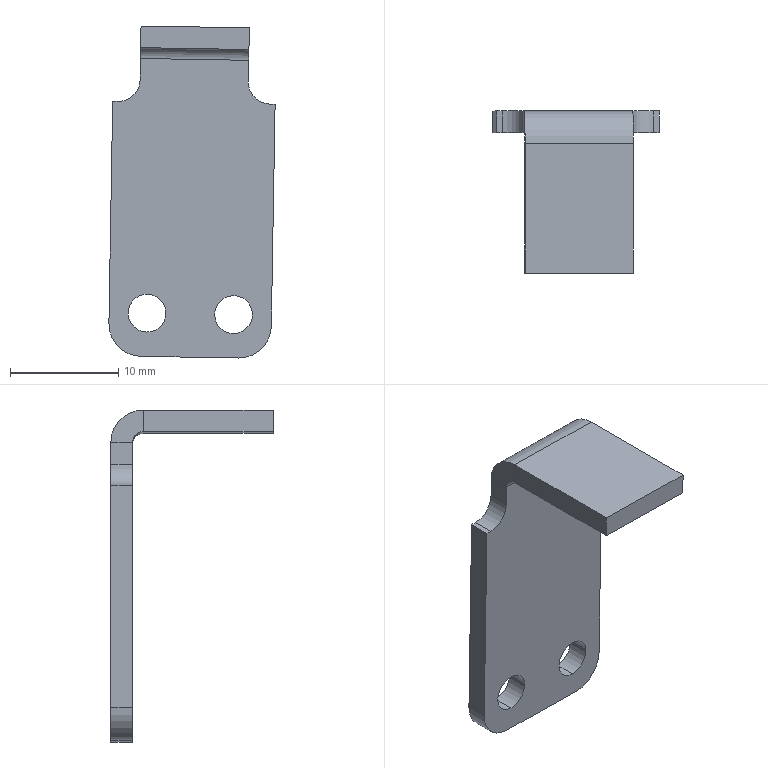Component | SolidWorks | RR40-1_InductionPlate-1 | 1 solid | 26 faces | box 15.35 x 15 x 30.66 mm | volume 1045 mm3 | plane 16 | cylinder 10 | commonest cylinder face diameters 3.5 x4 6 x3 4 x2 2 x1
STEP:
#1=COLOUR_RGB('',0.7922,0.8196,0.9333);
#2=FILL_AREA_STYLE_COLOUR('',#1);
#3=FILL_AREA_STYLE('',(#2));
#4=SURFACE_STYLE_FILL_AREA(#3);
#5=SURFACE_SIDE_STYLE('',(#4));
#6=SURFACE_STYLE_USAGE(.BOTH.,#5);
#7=PRESENTATION_STYLE_ASSIGNMENT((#6));
#8=CARTESIAN_POINT('',(22.955,37.638,-80.989));
#9=VERTEX_POINT('',#8);
#10=CARTESIAN_POINT('',(22.952,37.638,-81.127));
#11=VERTEX_POINT('',#10);
#12=CARTESIAN_POINT('',(22.953,37.638,-81.058));
#13=DIRECTION('',(-0.,-1.,-0.));
#14=DIRECTION('',(-0.01698,0.,-0.9999));
#15=AXIS2_PLACEMENT_3D('',#12,#13,#14);
#16=CIRCLE('',#15,0.0689);
#17=EDGE_CURVE('',#9,#11,#16,.T.);
#18=ORIENTED_EDGE('',*,*,#17,.T.);
#19=CARTESIAN_POINT('',(22.952,37.717,-81.127));
#20=VERTEX_POINT('',#19);
#21=CARTESIAN_POINT('',(22.952,37.717,-81.127));
#22=DIRECTION('',(0.,1.,0.));
#23=VECTOR('',#22,39.37);
#24=LINE('',#21,#23);
#25=EDGE_CURVE('',#11,#20,#24,.T.);
#26=ORIENTED_EDGE('',*,*,#25,.T.);
#27=CARTESIAN_POINT('',(22.955,37.717,-80.989));
#28=VERTEX_POINT('',#27);
#29=CARTESIAN_POINT('',(22.953,37.717,-81.058));
#30=DIRECTION('',(0.,1.,0.));
#31=DIRECTION('',(0.01698,0.,0.9999));
#32=AXIS2_PLACEMENT_3D('',#29,#30,#31);
#33=CIRCLE('',#32,0.0689);
#34=EDGE_CURVE('',#20,#28,#33,.T.);
#35=ORIENTED_EDGE('',*,*,#34,.T.);
#36=CARTESIAN_POINT('',(22.955,37.717,-80.989));
#37=DIRECTION('',(0.,1.,0.));
#38=VECTOR('',#37,39.37);
#39=LINE('',#36,#38);
#40=EDGE_CURVE('',#9,#28,#39,.T.);
#41=ORIENTED_EDGE('',*,*,#40,.F.);
#42=EDGE_LOOP('',(#18,#26,#35,#41));
#43=FACE_OUTER_BOUND('',#42,.T.);
#44=CARTESIAN_POINT('',(22.953,37.717,-81.058));
#45=DIRECTION('',(0.,1.,0.));
#46=DIRECTION('',(0.01698,0.,0.9999));
#47=AXIS2_PLACEMENT_3D('',#44,#45,#46);
#48=CYLINDRICAL_SURFACE('',#47,0.0689);
#49=ADVANCED_FACE('',(#43),#48,.F.);
#50=CARTESIAN_POINT('',(23.269,37.638,-80.994));
#51=VERTEX_POINT('',#50);
#52=CARTESIAN_POINT('',(23.267,37.638,-81.132));
#53=VERTEX_POINT('',#52);
#54=CARTESIAN_POINT('',(23.268,37.638,-81.063));
#55=DIRECTION('',(-0.,-1.,-0.));
#56=DIRECTION('',(-0.01698,0.,-0.9999));
#57=AXIS2_PLACEMENT_3D('',#54,#55,#56);
#58=CIRCLE('',#57,0.0689);
#59=EDGE_CURVE('',#51,#53,#58,.T.);
#60=ORIENTED_EDGE('',*,*,#59,.T.);
#61=CARTESIAN_POINT('',(23.267,37.717,-81.132));
#62=VERTEX_POINT('',#61);
#63=CARTESIAN_POINT('',(23.267,37.717,-81.132));
#64=DIRECTION('',(0.,1.,0.));
#65=VECTOR('',#64,39.37);
#66=LINE('',#63,#65);
#67=EDGE_CURVE('',#53,#62,#66,.T.);
#68=ORIENTED_EDGE('',*,*,#67,.T.);
#69=CARTESIAN_POINT('',(23.269,37.717,-80.994));
#70=VERTEX_POINT('',#69);
#71=CARTESIAN_POINT('',(23.268,37.717,-81.063));
#72=DIRECTION('',(0.,1.,0.));
#73=DIRECTION('',(0.01698,0.,0.9999));
#74=AXIS2_PLACEMENT_3D('',#71,#72,#73);
#75=CIRCLE('',#74,0.0689);
#76=EDGE_CURVE('',#62,#70,#75,.T.);
#77=ORIENTED_EDGE('',*,*,#76,.T.);
#78=CARTESIAN_POINT('',(23.269,37.717,-80.994));
#79=DIRECTION('',(0.,1.,0.));
#80=VECTOR('',#79,39.37);
#81=LINE('',#78,#80);
#82=EDGE_CURVE('',#51,#70,#81,.T.);
#83=ORIENTED_EDGE('',*,*,#82,.F.);
#84=EDGE_LOOP('',(#60,#68,#77,#83));
#85=FACE_OUTER_BOUND('',#84,.T.);
#86=CARTESIAN_POINT('',(23.268,37.717,-81.063));
#87=DIRECTION('',(0.,1.,0.));
#88=DIRECTION('',(0.01698,0.,0.9999));
#89=AXIS2_PLACEMENT_3D('',#86,#87,#88);
#90=CYLINDRICAL_SURFACE('',#89,0.0689);
#91=ADVANCED_FACE('',(#85),#90,.F.);
#92=CARTESIAN_POINT('',(23.323,37.638,-80.139));
#93=VERTEX_POINT('',#92);
#94=CARTESIAN_POINT('',(23.322,37.638,-80.218));
#95=VERTEX_POINT('',#94);
#96=CARTESIAN_POINT('',(23.305,37.638,-81.221));
#97=DIRECTION('',(-0.01698,0.,-0.9999));
#98=VECTOR('',#97,39.37);
#99=LINE('',#96,#98);
#100=EDGE_CURVE('',#93,#95,#99,.T.);
#101=ORIENTED_EDGE('',*,*,#100,.T.);
#102=CARTESIAN_POINT('',(23.322,37.717,-80.218));
#103=VERTEX_POINT('',#102);
#104=CARTESIAN_POINT('',(23.322,37.126,-80.218));
#105=DIRECTION('',(0.,1.,0.));
#106=VECTOR('',#105,39.37);
#107=LINE('',#104,#106);
#108=EDGE_CURVE('',#95,#103,#107,.T.);
#109=ORIENTED_EDGE('',*,*,#108,.T.);
#110=CARTESIAN_POINT('',(23.323,37.717,-80.139));
#111=VERTEX_POINT('',#110);
#112=CARTESIAN_POINT('',(23.321,37.717,-80.296));
#113=DIRECTION('',(0.01698,-0.,0.9999));
#114=VECTOR('',#113,39.37);
#115=LINE('',#112,#114);
#116=EDGE_CURVE('',#103,#111,#115,.T.);
#117=ORIENTED_EDGE('',*,*,#116,.T.);
#118=CARTESIAN_POINT('',(23.323,37.717,-80.139));
#119=DIRECTION('',(0.,-1.,0.));
#120=VECTOR('',#119,39.37);
#121=LINE('',#118,#120);
#122=EDGE_CURVE('',#111,#93,#121,.T.);
#123=ORIENTED_EDGE('',*,*,#122,.T.);
#124=EDGE_LOOP('',(#101,#109,#117,#123));
#125=FACE_OUTER_BOUND('',#124,.T.);
#126=CARTESIAN_POINT('',(23.321,37.126,-80.296));
#127=DIRECTION('',(-0.9999,0.,0.01698));
#128=DIRECTION('',(0.01698,0.,0.9999));
#129=AXIS2_PLACEMENT_3D('',#126,#127,#128);
#130=PLANE('',#129);
#131=ADVANCED_FACE('',(#125),#130,.F.);
#132=CARTESIAN_POINT('',(23.324,37.126,-80.099));
#133=VERTEX_POINT('',#132);
#134=CARTESIAN_POINT('',(23.324,37.598,-80.099));
#135=VERTEX_POINT('',#134);
#136=CARTESIAN_POINT('',(23.324,37.598,-80.099));
#137=DIRECTION('',(0.,1.,-0.));
#138=VECTOR('',#137,39.37);
#139=LINE('',#136,#138);
#140=EDGE_CURVE('',#133,#135,#139,.T.);
#141=ORIENTED_EDGE('',*,*,#140,.T.);
#142=CARTESIAN_POINT('',(23.325,37.598,-80.021));
#143=VERTEX_POINT('',#142);
#144=CARTESIAN_POINT('',(23.324,37.598,-80.099));
#145=DIRECTION('',(0.01698,0.,0.9999));
#146=VECTOR('',#145,39.37);
#147=LINE('',#144,#146);
#148=EDGE_CURVE('',#135,#143,#147,.T.);
#149=ORIENTED_EDGE('',*,*,#148,.T.);
#150=CARTESIAN_POINT('',(23.325,37.126,-80.021));
#151=VERTEX_POINT('',#150);
#152=CARTESIAN_POINT('',(23.325,37.598,-80.021));
#153=DIRECTION('',(0.,1.,-0.));
#154=VECTOR('',#153,39.37);
#155=LINE('',#152,#154);
#156=EDGE_CURVE('',#151,#143,#155,.T.);
#157=ORIENTED_EDGE('',*,*,#156,.F.);
#158=CARTESIAN_POINT('',(23.321,37.126,-80.296));
#159=DIRECTION('',(0.01698,-0.,0.9999));
#160=VECTOR('',#159,39.37);
#161=LINE('',#158,#160);
#162=EDGE_CURVE('',#133,#151,#161,.T.);
#163=ORIENTED_EDGE('',*,*,#162,.F.);
#164=EDGE_LOOP('',(#141,#149,#157,#163));
#165=FACE_OUTER_BOUND('',#164,.T.);
#166=CARTESIAN_POINT('',(23.321,37.126,-80.296));
#167=DIRECTION('',(-0.9999,0.,0.01698));
#168=DIRECTION('',(0.01698,0.,0.9999));
#169=AXIS2_PLACEMENT_3D('',#166,#167,#168);
#170=PLANE('',#169);
#171=ADVANCED_FACE('',(#165),#170,.F.);
#172=CARTESIAN_POINT('',(22.928,37.717,-80.211));
#173=VERTEX_POINT('',#172);
#174=CARTESIAN_POINT('',(22.93,37.717,-80.132));
#175=VERTEX_POINT('',#174);
#176=CARTESIAN_POINT('',(22.911,37.717,-81.215));
#177=DIRECTION('',(0.01698,-0.,0.9999));
#178=VECTOR('',#177,39.37);
#179=LINE('',#176,#178);
#180=EDGE_CURVE('',#173,#175,#179,.T.);
#181=ORIENTED_EDGE('',*,*,#180,.F.);
#182=CARTESIAN_POINT('',(22.928,37.638,-80.211));
#183=VERTEX_POINT('',#182);
#184=CARTESIAN_POINT('',(22.928,37.126,-80.211));
#185=DIRECTION('',(-0.,-1.,-0.));
#186=VECTOR('',#185,39.37);
#187=LINE('',#184,#186);
#188=EDGE_CURVE('',#173,#183,#187,.T.);
#189=ORIENTED_EDGE('',*,*,#188,.T.);
#190=CARTESIAN_POINT('',(22.93,37.638,-80.132));
#191=VERTEX_POINT('',#190);
#192=CARTESIAN_POINT('',(22.911,37.638,-81.215));
#193=DIRECTION('',(-0.01698,0.,-0.9999));
#194=VECTOR('',#193,39.37);
#195=LINE('',#192,#194);
#196=EDGE_CURVE('',#191,#183,#195,.T.);
#197=ORIENTED_EDGE('',*,*,#196,.F.);
#198=CARTESIAN_POINT('',(22.93,37.638,-80.132));
#199=DIRECTION('',(0.,1.,-0.));
#200=VECTOR('',#199,39.37);
#201=LINE('',#198,#200);
#202=EDGE_CURVE('',#191,#175,#201,.T.);
#203=ORIENTED_EDGE('',*,*,#202,.T.);
#204=EDGE_LOOP('',(#181,#189,#197,#203));
#205=FACE_OUTER_BOUND('',#204,.T.);
#206=CARTESIAN_POINT('',(22.911,37.126,-81.215));
#207=DIRECTION('',(-0.9999,0.,0.01698));
#208=DIRECTION('',(0.01698,0.,0.9999));
#209=AXIS2_PLACEMENT_3D('',#206,#207,#208);
#210=PLANE('',#209);
#211=ADVANCED_FACE('',(#205),#210,.T.);
#212=CARTESIAN_POINT('',(22.932,37.126,-80.014));
#213=VERTEX_POINT('',#212);
#214=CARTESIAN_POINT('',(22.932,37.598,-80.014));
#215=VERTEX_POINT('',#214);
#216=CARTESIAN_POINT('',(22.932,37.598,-80.014));
#217=DIRECTION('',(0.,1.,-0.));
#218=VECTOR('',#217,39.37);
#219=LINE('',#216,#218);
#220=EDGE_CURVE('',#213,#215,#219,.T.);
#221=ORIENTED_EDGE('',*,*,#220,.T.);
#222=CARTESIAN_POINT('',(22.93,37.598,-80.093));
#223=VERTEX_POINT('',#222);
#224=CARTESIAN_POINT('',(22.932,37.598,-80.014));
#225=DIRECTION('',(-0.01698,-0.,-0.9999));
#226=VECTOR('',#225,39.37);
#227=LINE('',#224,#226);
#228=EDGE_CURVE('',#215,#223,#227,.T.);
#229=ORIENTED_EDGE('',*,*,#228,.T.);
#230=CARTESIAN_POINT('',(22.93,37.126,-80.093));
#231=VERTEX_POINT('',#230);
#232=CARTESIAN_POINT('',(22.93,37.598,-80.093));
#233=DIRECTION('',(0.,1.,-0.));
#234=VECTOR('',#233,39.37);
#235=LINE('',#232,#234);
#236=EDGE_CURVE('',#231,#223,#235,.T.);
#237=ORIENTED_EDGE('',*,*,#236,.F.);
#238=CARTESIAN_POINT('',(22.911,37.126,-81.215));
#239=DIRECTION('',(0.01698,-0.,0.9999));
#240=VECTOR('',#239,39.37);
#241=LINE('',#238,#240);
#242=EDGE_CURVE('',#231,#213,#241,.T.);
#243=ORIENTED_EDGE('',*,*,#242,.T.);
#244=EDGE_LOOP('',(#221,#229,#237,#243));
#245=FACE_OUTER_BOUND('',#244,.T.);
#246=CARTESIAN_POINT('',(22.911,37.126,-81.215));
#247=DIRECTION('',(-0.9999,0.,0.01698));
#248=DIRECTION('',(0.01698,0.,0.9999));
#249=AXIS2_PLACEMENT_3D('',#246,#247,#248);
#250=PLANE('',#249);
#251=ADVANCED_FACE('',(#245),#250,.T.);
#252=ORIENTED_EDGE('',*,*,#17,.F.);
#253=CARTESIAN_POINT('',(22.953,37.638,-81.058));
#254=DIRECTION('',(-0.,-1.,-0.));
#255=DIRECTION('',(-0.01698,0.,-0.9999));
#256=AXIS2_PLACEMENT_3D('',#253,#254,#255);
#257=CIRCLE('',#256,0.0689);
#258=EDGE_CURVE('',#11,#9,#257,.T.);
#259=ORIENTED_EDGE('',*,*,#258,.F.);
#260=EDGE_LOOP('',(#252,#259));
#261=FACE_BOUND('',#260,.T.);
#262=ORIENTED_EDGE('',*,*,#59,.F.);
#263=CARTESIAN_POINT('',(23.268,37.638,-81.063));
#264=DIRECTION('',(-0.,-1.,-0.));
#265=DIRECTION('',(-0.01698,0.,-0.9999));
#266=AXIS2_PLACEMENT_3D('',#263,#264,#265);
#267=CIRCLE('',#266,0.0689);
#268=EDGE_CURVE('',#53,#51,#267,.T.);
#269=ORIENTED_EDGE('',*,*,#268,.F.);
#270=EDGE_LOOP('',(#262,#269));
#271=FACE_BOUND('',#270,.T.);
#272=CARTESIAN_POINT('',(23.405,37.638,-81.105));
#273=VERTEX_POINT('',#272);
#274=CARTESIAN_POINT('',(23.419,37.638,-80.298));
#275=VERTEX_POINT('',#274);
#276=CARTESIAN_POINT('',(23.403,37.638,-81.223));
#277=DIRECTION('',(0.01698,-0.,0.9999));
#278=VECTOR('',#277,39.37);
#279=LINE('',#276,#278);
#280=EDGE_CURVE('',#273,#275,#279,.T.);
#281=ORIENTED_EDGE('',*,*,#280,.T.);
#282=CARTESIAN_POINT('',(23.399,37.638,-80.298));
#283=VERTEX_POINT('',#282);
#284=CARTESIAN_POINT('',(23.419,37.638,-80.298));
#285=DIRECTION('',(-0.9999,0.,0.01698));
#286=VECTOR('',#285,39.37);
#287=LINE('',#284,#286);
#288=EDGE_CURVE('',#275,#283,#287,.T.);
#289=ORIENTED_EDGE('',*,*,#288,.T.);
#290=CARTESIAN_POINT('',(23.401,37.638,-80.219));
#291=DIRECTION('',(0.,1.,0.));
#292=DIRECTION('',(-0.01698,0.,-0.9999));
#293=AXIS2_PLACEMENT_3D('',#290,#291,#292);
#294=CIRCLE('',#293,0.07874);
#295=EDGE_CURVE('',#283,#95,#294,.T.);
#296=ORIENTED_EDGE('',*,*,#295,.T.);
#297=ORIENTED_EDGE('',*,*,#100,.F.);
#298=CARTESIAN_POINT('',(23.422,37.638,-80.141));
#299=DIRECTION('',(-0.9999,0.,0.01698));
#300=VECTOR('',#299,39.37);
#301=LINE('',#298,#300);
#302=EDGE_CURVE('',#93,#191,#301,.T.);
#303=ORIENTED_EDGE('',*,*,#302,.T.);
#304=ORIENTED_EDGE('',*,*,#196,.T.);
#305=CARTESIAN_POINT('',(22.848,37.638,-80.288));
#306=VERTEX_POINT('',#305);
#307=CARTESIAN_POINT('',(22.85,37.638,-80.21));
#308=DIRECTION('',(0.,1.,0.));
#309=DIRECTION('',(-0.01698,0.,-0.9999));
#310=AXIS2_PLACEMENT_3D('',#307,#308,#309);
#311=CIRCLE('',#310,0.07874);
#312=EDGE_CURVE('',#183,#306,#311,.T.);
#313=ORIENTED_EDGE('',*,*,#312,.T.);
#314=CARTESIAN_POINT('',(22.829,37.638,-80.288));
#315=VERTEX_POINT('',#314);
#316=CARTESIAN_POINT('',(23.419,37.638,-80.298));
#317=DIRECTION('',(0.9999,-0.,-0.01698));
#318=VECTOR('',#317,39.37);
#319=LINE('',#316,#318);
#320=EDGE_CURVE('',#315,#306,#319,.T.);
#321=ORIENTED_EDGE('',*,*,#320,.F.);
#322=CARTESIAN_POINT('',(22.815,37.638,-81.095));
#323=VERTEX_POINT('',#322);
#324=CARTESIAN_POINT('',(22.813,37.638,-81.213));
#325=DIRECTION('',(0.01698,-0.,0.9999));
#326=VECTOR('',#325,39.37);
#327=LINE('',#324,#326);
#328=EDGE_CURVE('',#323,#315,#327,.T.);
#329=ORIENTED_EDGE('',*,*,#328,.F.);
#330=CARTESIAN_POINT('',(22.931,37.638,-81.215));
#331=VERTEX_POINT('',#330);
#332=CARTESIAN_POINT('',(22.933,37.638,-81.097));
#333=DIRECTION('',(-0.,-1.,-0.));
#334=DIRECTION('',(-0.01698,0.,-0.9999));
#335=AXIS2_PLACEMENT_3D('',#332,#333,#334);
#336=CIRCLE('',#335,0.1181);
#337=EDGE_CURVE('',#323,#331,#336,.T.);
#338=ORIENTED_EDGE('',*,*,#337,.T.);
#339=CARTESIAN_POINT('',(23.285,37.638,-81.221));
#340=VERTEX_POINT('',#339);
#341=CARTESIAN_POINT('',(23.403,37.638,-81.223));
#342=DIRECTION('',(-0.9999,0.,0.01698));
#343=VECTOR('',#342,39.37);
#344=LINE('',#341,#343);
#345=EDGE_CURVE('',#340,#331,#344,.T.);
#346=ORIENTED_EDGE('',*,*,#345,.F.);
#347=CARTESIAN_POINT('',(23.287,37.638,-81.103));
#348=DIRECTION('',(-0.,-1.,-0.));
#349=DIRECTION('',(-0.01698,0.,-0.9999));
#350=AXIS2_PLACEMENT_3D('',#347,#348,#349);
#351=CIRCLE('',#350,0.1181);
#352=EDGE_CURVE('',#340,#273,#351,.T.);
#353=ORIENTED_EDGE('',*,*,#352,.T.);
#354=EDGE_LOOP('',(#281,#289,#296,#297,#303,#304,#313,#321,#329,#338,#346,#353));
#355=FACE_OUTER_BOUND('',#354,.T.);
#356=CARTESIAN_POINT('',(23.403,37.638,-81.223));
#357=DIRECTION('',(-0.,-1.,-0.));
#358=DIRECTION('',(-0.01698,0.,-0.9999));
#359=AXIS2_PLACEMENT_3D('',#356,#357,#358);
#360=PLANE('',#359);
#361=ADVANCED_FACE('',(#261,#271,#355),#360,.T.);
#362=CARTESIAN_POINT('',(22.953,37.717,-81.058));
#363=DIRECTION('',(0.,1.,0.));
#364=DIRECTION('',(0.01698,0.,0.9999));
#365=AXIS2_PLACEMENT_3D('',#362,#363,#364);
#366=CIRCLE('',#365,0.0689);
#367=EDGE_CURVE('',#28,#20,#366,.T.);
#368=ORIENTED_EDGE('',*,*,#367,.F.);
#369=ORIENTED_EDGE('',*,*,#34,.F.);
#370=EDGE_LOOP('',(#368,#369));
#371=FACE_BOUND('',#370,.T.);
#372=CARTESIAN_POINT('',(23.268,37.717,-81.063));
#373=DIRECTION('',(0.,1.,0.));
#374=DIRECTION('',(0.01698,0.,0.9999));
#375=AXIS2_PLACEMENT_3D('',#372,#373,#374);
#376=CIRCLE('',#375,0.0689);
#377=EDGE_CURVE('',#70,#62,#376,.T.);
#378=ORIENTED_EDGE('',*,*,#377,.F.);
#379=ORIENTED_EDGE('',*,*,#76,.F.);
#380=EDGE_LOOP('',(#378,#379));
#381=FACE_BOUND('',#380,.T.);
#382=ORIENTED_EDGE('',*,*,#116,.F.);
#383=CARTESIAN_POINT('',(23.399,37.717,-80.298));
#384=VERTEX_POINT('',#383);
#385=CARTESIAN_POINT('',(23.401,37.717,-80.219));
#386=DIRECTION('',(-0.,-1.,-0.));
#387=DIRECTION('',(-0.01698,0.,-0.9999));
#388=AXIS2_PLACEMENT_3D('',#385,#386,#387);
#389=CIRCLE('',#388,0.07874);
#390=EDGE_CURVE('',#103,#384,#389,.T.);
#391=ORIENTED_EDGE('',*,*,#390,.T.);
#392=CARTESIAN_POINT('',(23.419,37.717,-80.298));
#393=VERTEX_POINT('',#392);
#394=CARTESIAN_POINT('',(23.321,37.717,-80.296));
#395=DIRECTION('',(0.9999,-0.,-0.01698));
#396=VECTOR('',#395,39.37);
#397=LINE('',#394,#396);
#398=EDGE_CURVE('',#384,#393,#397,.T.);
#399=ORIENTED_EDGE('',*,*,#398,.T.);
#400=CARTESIAN_POINT('',(23.405,37.717,-81.105));
#401=VERTEX_POINT('',#400);
#402=CARTESIAN_POINT('',(23.403,37.717,-81.223));
#403=DIRECTION('',(0.01698,-0.,0.9999));
#404=VECTOR('',#403,39.37);
#405=LINE('',#402,#404);
#406=EDGE_CURVE('',#401,#393,#405,.T.);
#407=ORIENTED_EDGE('',*,*,#406,.F.);
#408=CARTESIAN_POINT('',(23.285,37.717,-81.221));
#409=VERTEX_POINT('',#408);
#410=CARTESIAN_POINT('',(23.287,37.717,-81.103));
#411=DIRECTION('',(0.,1.,0.));
#412=DIRECTION('',(-0.01698,0.,-0.9999));
#413=AXIS2_PLACEMENT_3D('',#410,#411,#412);
#414=CIRCLE('',#413,0.1181);
#415=EDGE_CURVE('',#401,#409,#414,.T.);
#416=ORIENTED_EDGE('',*,*,#415,.T.);
#417=CARTESIAN_POINT('',(22.931,37.717,-81.215));
#418=VERTEX_POINT('',#417);
#419=CARTESIAN_POINT('',(23.403,37.717,-81.223));
#420=DIRECTION('',(-0.9999,0.,0.01698));
#421=VECTOR('',#420,39.37);
#422=LINE('',#419,#421);
#423=EDGE_CURVE('',#409,#418,#422,.T.);
#424=ORIENTED_EDGE('',*,*,#423,.T.);
#425=CARTESIAN_POINT('',(22.815,37.717,-81.095));
#426=VERTEX_POINT('',#425);
#427=CARTESIAN_POINT('',(22.933,37.717,-81.097));
#428=DIRECTION('',(0.,1.,0.));
#429=DIRECTION('',(-0.01698,0.,-0.9999));
#430=AXIS2_PLACEMENT_3D('',#427,#428,#429);
#431=CIRCLE('',#430,0.1181);
#432=EDGE_CURVE('',#418,#426,#431,.T.);
#433=ORIENTED_EDGE('',*,*,#432,.T.);
#434=CARTESIAN_POINT('',(22.829,37.717,-80.288));
#435=VERTEX_POINT('',#434);
#436=CARTESIAN_POINT('',(22.813,37.717,-81.213));
#437=DIRECTION('',(0.01698,-0.,0.9999));
#438=VECTOR('',#437,39.37);
#439=LINE('',#436,#438);
#440=EDGE_CURVE('',#426,#435,#439,.T.);
#441=ORIENTED_EDGE('',*,*,#440,.T.);
#442=CARTESIAN_POINT('',(22.848,37.717,-80.288));
#443=VERTEX_POINT('',#442);
#444=CARTESIAN_POINT('',(23.124,37.717,-80.293));
#445=DIRECTION('',(-0.9999,0.,0.01698));
#446=VECTOR('',#445,39.37);
#447=LINE('',#444,#446);
#448=EDGE_CURVE('',#443,#435,#447,.T.);
#449=ORIENTED_EDGE('',*,*,#448,.F.);
#450=CARTESIAN_POINT('',(22.85,37.717,-80.21));
#451=DIRECTION('',(-0.,-1.,-0.));
#452=DIRECTION('',(-0.01698,0.,-0.9999));
#453=AXIS2_PLACEMENT_3D('',#450,#451,#452);
#454=CIRCLE('',#453,0.07874);
#455=EDGE_CURVE('',#443,#173,#454,.T.);
#456=ORIENTED_EDGE('',*,*,#455,.T.);
#457=ORIENTED_EDGE('',*,*,#180,.T.);
#458=CARTESIAN_POINT('',(23.422,37.717,-80.141));
#459=DIRECTION('',(-0.9999,0.,0.01698));
#460=VECTOR('',#459,39.37);
#461=LINE('',#458,#460);
#462=EDGE_CURVE('',#111,#175,#461,.T.);
#463=ORIENTED_EDGE('',*,*,#462,.F.);
#464=EDGE_LOOP('',(#382,#391,#399,#407,#416,#424,#433,#441,#449,#456,#457,#463));
#465=FACE_OUTER_BOUND('',#464,.T.);
#466=CARTESIAN_POINT('',(23.403,37.717,-81.223));
#467=DIRECTION('',(-0.,-1.,-0.));
#468=DIRECTION('',(-0.01698,0.,-0.9999));
#469=AXIS2_PLACEMENT_3D('',#466,#467,#468);
#470=PLANE('',#469);
#471=ADVANCED_FACE('',(#371,#381,#465),#470,.F.);
#472=ORIENTED_EDGE('',*,*,#406,.T.);
#473=CARTESIAN_POINT('',(23.419,37.598,-80.298));
#474=DIRECTION('',(-0.,-1.,-0.));
#475=VECTOR('',#474,39.37);
#476=LINE('',#473,#475);
#477=EDGE_CURVE('',#393,#275,#476,.T.);
#478=ORIENTED_EDGE('',*,*,#477,.T.);
#479=ORIENTED_EDGE('',*,*,#280,.F.);
#480=CARTESIAN_POINT('',(23.405,37.598,-81.105));
#481=DIRECTION('',(0.,1.,0.));
#482=VECTOR('',#481,39.37);
#483=LINE('',#480,#482);
#484=EDGE_CURVE('',#273,#401,#483,.T.);
#485=ORIENTED_EDGE('',*,*,#484,.T.);
#486=EDGE_LOOP('',(#472,#478,#479,#485));
#487=FACE_OUTER_BOUND('',#486,.T.);
#488=CARTESIAN_POINT('',(23.422,37.598,-80.101));
#489=DIRECTION('',(0.9999,-0.,-0.01698));
#490=DIRECTION('',(-0.01698,-0.,-0.9999));
#491=AXIS2_PLACEMENT_3D('',#488,#489,#490);
#492=PLANE('',#491);
#493=ADVANCED_FACE('',(#487),#492,.T.);
#494=CARTESIAN_POINT('',(23.424,37.126,-80.022));
#495=DIRECTION('',(-0.9999,0.,0.01698));
#496=VECTOR('',#495,39.37);
#497=LINE('',#494,#496);
#498=EDGE_CURVE('',#151,#213,#497,.T.);
#499=ORIENTED_EDGE('',*,*,#498,.F.);
#500=ORIENTED_EDGE('',*,*,#156,.T.);
#501=CARTESIAN_POINT('',(23.424,37.598,-80.022));
#502=DIRECTION('',(-0.9999,0.,0.01698));
#503=VECTOR('',#502,39.37);
#504=LINE('',#501,#503);
#505=EDGE_CURVE('',#143,#215,#504,.T.);
#506=ORIENTED_EDGE('',*,*,#505,.T.);
#507=ORIENTED_EDGE('',*,*,#220,.F.);
#508=EDGE_LOOP('',(#499,#500,#506,#507));
#509=FACE_OUTER_BOUND('',#508,.T.);
#510=CARTESIAN_POINT('',(23.424,37.598,-80.022));
#511=DIRECTION('',(-0.01698,-0.,-0.9999));
#512=DIRECTION('',(-0.9999,0.,0.01698));
#513=AXIS2_PLACEMENT_3D('',#510,#511,#512);
#514=PLANE('',#513);
#515=ADVANCED_FACE('',(#509),#514,.F.);
#516=ORIENTED_EDGE('',*,*,#162,.T.);
#517=ORIENTED_EDGE('',*,*,#498,.T.);
#518=ORIENTED_EDGE('',*,*,#242,.F.);
#519=CARTESIAN_POINT('',(23.422,37.126,-80.101));
#520=DIRECTION('',(-0.9999,0.,0.01698));
#521=VECTOR('',#520,39.37);
#522=LINE('',#519,#521);
#523=EDGE_CURVE('',#133,#231,#522,.T.);
#524=ORIENTED_EDGE('',*,*,#523,.F.);
#525=EDGE_LOOP('',(#516,#517,#518,#524));
#526=FACE_OUTER_BOUND('',#525,.T.);
#527=CARTESIAN_POINT('',(23.422,37.126,-80.101));
#528=DIRECTION('',(-0.,-1.,0.));
#529=DIRECTION('',(-0.01698,-0.,-0.9999));
#530=AXIS2_PLACEMENT_3D('',#527,#528,#529);
#531=PLANE('',#530);
#532=ADVANCED_FACE('',(#526),#531,.T.);
#533=ORIENTED_EDGE('',*,*,#140,.F.);
#534=ORIENTED_EDGE('',*,*,#523,.T.);
#535=ORIENTED_EDGE('',*,*,#236,.T.);
#536=CARTESIAN_POINT('',(23.422,37.598,-80.101));
#537=DIRECTION('',(-0.9999,0.,0.01698));
#538=VECTOR('',#537,39.37);
#539=LINE('',#536,#538);
#540=EDGE_CURVE('',#135,#223,#539,.T.);
#541=ORIENTED_EDGE('',*,*,#540,.F.);
#542=EDGE_LOOP('',(#533,#534,#535,#541));
#543=FACE_OUTER_BOUND('',#542,.T.);
#544=CARTESIAN_POINT('',(23.422,37.598,-80.101));
#545=DIRECTION('',(-0.01698,-0.,-0.9999));
#546=DIRECTION('',(-0.9999,0.,0.01698));
#547=AXIS2_PLACEMENT_3D('',#544,#545,#546);
#548=PLANE('',#547);
#549=ADVANCED_FACE('',(#543),#548,.T.);
#550=CARTESIAN_POINT('',(23.323,37.598,-80.139));
#551=DIRECTION('',(-0.9999,0.,0.01698));
#552=DIRECTION('',(0.01698,0.,0.9999));
#553=AXIS2_PLACEMENT_3D('',#550,#551,#552);
#554=CIRCLE('',#553,0.03937);
#555=EDGE_CURVE('',#135,#93,#554,.T.);
#556=ORIENTED_EDGE('',*,*,#555,.F.);
#557=ORIENTED_EDGE('',*,*,#540,.T.);
#558=CARTESIAN_POINT('',(22.93,37.598,-80.132));
#559=DIRECTION('',(-0.9999,0.,0.01698));
#560=DIRECTION('',(0.01698,0.,0.9999));
#561=AXIS2_PLACEMENT_3D('',#558,#559,#560);
#562=CIRCLE('',#561,0.03937);
#563=EDGE_CURVE('',#223,#191,#562,.T.);
#564=ORIENTED_EDGE('',*,*,#563,.T.);
#565=ORIENTED_EDGE('',*,*,#302,.F.);
#566=EDGE_LOOP('',(#556,#557,#564,#565));
#567=FACE_OUTER_BOUND('',#566,.T.);
#568=CARTESIAN_POINT('',(23.422,37.598,-80.141));
#569=DIRECTION('',(-0.9999,0.,0.01698));
#570=DIRECTION('',(0.01698,0.,0.9999));
#571=AXIS2_PLACEMENT_3D('',#568,#569,#570);
#572=CYLINDRICAL_SURFACE('',#571,0.03937);
#573=ADVANCED_FACE('',(#567),#572,.F.);
#574=ORIENTED_EDGE('',*,*,#505,.F.);
#575=CARTESIAN_POINT('',(23.323,37.598,-80.139));
#576=DIRECTION('',(-0.9999,0.,0.01698));
#577=DIRECTION('',(0.01698,0.,0.9999));
#578=AXIS2_PLACEMENT_3D('',#575,#576,#577);
#579=CIRCLE('',#578,0.1181);
#580=EDGE_CURVE('',#143,#111,#579,.T.);
#581=ORIENTED_EDGE('',*,*,#580,.T.);
#582=ORIENTED_EDGE('',*,*,#462,.T.);
#583=CARTESIAN_POINT('',(22.93,37.598,-80.132));
#584=DIRECTION('',(-0.9999,0.,0.01698));
#585=DIRECTION('',(0.01698,0.,0.9999));
#586=AXIS2_PLACEMENT_3D('',#583,#584,#585);
#587=CIRCLE('',#586,0.1181);
#588=EDGE_CURVE('',#215,#175,#587,.T.);
#589=ORIENTED_EDGE('',*,*,#588,.F.);
#590=EDGE_LOOP('',(#574,#581,#582,#589));
#591=FACE_OUTER_BOUND('',#590,.T.);
#592=CARTESIAN_POINT('',(23.422,37.598,-80.141));
#593=DIRECTION('',(-0.9999,0.,0.01698));
#594=DIRECTION('',(0.01698,0.,0.9999));
#595=AXIS2_PLACEMENT_3D('',#592,#593,#594);
#596=CYLINDRICAL_SURFACE('',#595,0.1181);
#597=ADVANCED_FACE('',(#591),#596,.T.);
#598=ORIENTED_EDGE('',*,*,#345,.T.);
#599=CARTESIAN_POINT('',(22.931,37.717,-81.215));
#600=DIRECTION('',(0.,1.,0.));
#601=VECTOR('',#600,39.37);
#602=LINE('',#599,#601);
#603=EDGE_CURVE('',#331,#418,#602,.T.);
#604=ORIENTED_EDGE('',*,*,#603,.T.);
#605=ORIENTED_EDGE('',*,*,#423,.F.);
#606=CARTESIAN_POINT('',(23.285,37.717,-81.221));
#607=DIRECTION('',(-0.,-1.,-0.));
#608=VECTOR('',#607,39.37);
#609=LINE('',#606,#608);
#610=EDGE_CURVE('',#409,#340,#609,.T.);
#611=ORIENTED_EDGE('',*,*,#610,.T.);
#612=EDGE_LOOP('',(#598,#604,#605,#611));
#613=FACE_OUTER_BOUND('',#612,.T.);
#614=CARTESIAN_POINT('',(23.403,37.717,-81.223));
#615=DIRECTION('',(-0.01698,0.,-0.9999));
#616=DIRECTION('',(0.,1.,0.));
#617=AXIS2_PLACEMENT_3D('',#614,#615,#616);
#618=PLANE('',#617);
#619=ADVANCED_FACE('',(#613),#618,.T.);
#620=ORIENTED_EDGE('',*,*,#328,.T.);
#621=CARTESIAN_POINT('',(22.829,37.598,-80.288));
#622=DIRECTION('',(0.,1.,0.));
#623=VECTOR('',#622,39.37);
#624=LINE('',#621,#623);
#625=EDGE_CURVE('',#315,#435,#624,.T.);
#626=ORIENTED_EDGE('',*,*,#625,.T.);
#627=ORIENTED_EDGE('',*,*,#440,.F.);
#628=CARTESIAN_POINT('',(22.815,37.638,-81.095));
#629=DIRECTION('',(-0.,-1.,-0.));
#630=VECTOR('',#629,39.37);
#631=LINE('',#628,#630);
#632=EDGE_CURVE('',#426,#323,#631,.T.);
#633=ORIENTED_EDGE('',*,*,#632,.T.);
#634=EDGE_LOOP('',(#620,#626,#627,#633));
#635=FACE_OUTER_BOUND('',#634,.T.);
#636=CARTESIAN_POINT('',(22.831,37.598,-80.13));
#637=DIRECTION('',(0.9999,-0.,-0.01698));
#638=DIRECTION('',(-0.01698,-0.,-0.9999));
#639=AXIS2_PLACEMENT_3D('',#636,#637,#638);
#640=PLANE('',#639);
#641=ADVANCED_FACE('',(#635),#640,.F.);
#642=ORIENTED_EDGE('',*,*,#432,.F.);
#643=ORIENTED_EDGE('',*,*,#603,.F.);
#644=ORIENTED_EDGE('',*,*,#337,.F.);
#645=ORIENTED_EDGE('',*,*,#632,.F.);
#646=EDGE_LOOP('',(#642,#643,#644,#645));
#647=FACE_OUTER_BOUND('',#646,.T.);
#648=CARTESIAN_POINT('',(22.933,37.598,-81.097));
#649=DIRECTION('',(0.,1.,0.));
#650=DIRECTION('',(0.01698,0.,0.9999));
#651=AXIS2_PLACEMENT_3D('',#648,#649,#650);
#652=CYLINDRICAL_SURFACE('',#651,0.1181);
#653=ADVANCED_FACE('',(#647),#652,.T.);
#654=ORIENTED_EDGE('',*,*,#415,.F.);
#655=ORIENTED_EDGE('',*,*,#484,.F.);
#656=ORIENTED_EDGE('',*,*,#352,.F.);
#657=ORIENTED_EDGE('',*,*,#610,.F.);
#658=EDGE_LOOP('',(#654,#655,#656,#657));
#659=FACE_OUTER_BOUND('',#658,.T.);
#660=CARTESIAN_POINT('',(23.287,37.717,-81.103));
#661=DIRECTION('',(-0.,-1.,-0.));
#662=DIRECTION('',(-0.01698,0.,-0.9999));
#663=AXIS2_PLACEMENT_3D('',#660,#661,#662);
#664=CYLINDRICAL_SURFACE('',#663,0.1181);
#665=ADVANCED_FACE('',(#659),#664,.T.);
#666=ORIENTED_EDGE('',*,*,#67,.F.);
#667=ORIENTED_EDGE('',*,*,#268,.T.);
#668=ORIENTED_EDGE('',*,*,#82,.T.);
#669=ORIENTED_EDGE('',*,*,#377,.T.);
#670=EDGE_LOOP('',(#666,#667,#668,#669));
#671=FACE_OUTER_BOUND('',#670,.T.);
#672=CARTESIAN_POINT('',(23.268,37.717,-81.063));
#673=DIRECTION('',(0.,1.,0.));
#674=DIRECTION('',(0.01698,0.,0.9999));
#675=AXIS2_PLACEMENT_3D('',#672,#673,#674);
#676=CYLINDRICAL_SURFACE('',#675,0.0689);
#677=ADVANCED_FACE('',(#671),#676,.F.);
#678=ORIENTED_EDGE('',*,*,#25,.F.);
#679=ORIENTED_EDGE('',*,*,#258,.T.);
#680=ORIENTED_EDGE('',*,*,#40,.T.);
#681=ORIENTED_EDGE('',*,*,#367,.T.);
#682=EDGE_LOOP('',(#678,#679,#680,#681));
#683=FACE_OUTER_BOUND('',#682,.T.);
#684=CARTESIAN_POINT('',(22.953,37.717,-81.058));
#685=DIRECTION('',(0.,1.,0.));
#686=DIRECTION('',(0.01698,0.,0.9999));
#687=AXIS2_PLACEMENT_3D('',#684,#685,#686);
#688=CYLINDRICAL_SURFACE('',#687,0.0689);
#689=ADVANCED_FACE('',(#683),#688,.F.);
#690=ORIENTED_EDGE('',*,*,#202,.F.);
#691=ORIENTED_EDGE('',*,*,#563,.F.);
#692=ORIENTED_EDGE('',*,*,#228,.F.);
#693=ORIENTED_EDGE('',*,*,#588,.T.);
#694=EDGE_LOOP('',(#690,#691,#692,#693));
#695=FACE_OUTER_BOUND('',#694,.T.);
#696=CARTESIAN_POINT('',(22.911,37.126,-81.215));
#697=DIRECTION('',(-0.9999,0.,0.01698));
#698=DIRECTION('',(0.01698,0.,0.9999));
#699=AXIS2_PLACEMENT_3D('',#696,#697,#698);
#700=PLANE('',#699);
#701=ADVANCED_FACE('',(#695),#700,.T.);
#702=ORIENTED_EDGE('',*,*,#320,.T.);
#703=CARTESIAN_POINT('',(22.848,37.126,-80.288));
#704=DIRECTION('',(0.,1.,0.));
#705=VECTOR('',#704,39.37);
#706=LINE('',#703,#705);
#707=EDGE_CURVE('',#306,#443,#706,.T.);
#708=ORIENTED_EDGE('',*,*,#707,.T.);
#709=ORIENTED_EDGE('',*,*,#448,.T.);
#710=ORIENTED_EDGE('',*,*,#625,.F.);
#711=EDGE_LOOP('',(#702,#708,#709,#710));
#712=FACE_OUTER_BOUND('',#711,.T.);
#713=CARTESIAN_POINT('',(23.124,37.126,-80.293));
#714=DIRECTION('',(-0.01698,0.,-0.9999));
#715=DIRECTION('',(-0.9999,0.,0.01698));
#716=AXIS2_PLACEMENT_3D('',#713,#714,#715);
#717=PLANE('',#716);
#718=ADVANCED_FACE('',(#712),#717,.F.);
#719=ORIENTED_EDGE('',*,*,#122,.F.);
#720=ORIENTED_EDGE('',*,*,#580,.F.);
#721=ORIENTED_EDGE('',*,*,#148,.F.);
#722=ORIENTED_EDGE('',*,*,#555,.T.);
#723=EDGE_LOOP('',(#719,#720,#721,#722));
#724=FACE_OUTER_BOUND('',#723,.T.);
#725=CARTESIAN_POINT('',(23.321,37.126,-80.296));
#726=DIRECTION('',(-0.9999,0.,0.01698));
#727=DIRECTION('',(0.01698,0.,0.9999));
#728=AXIS2_PLACEMENT_3D('',#725,#726,#727);
#729=PLANE('',#728);
#730=ADVANCED_FACE('',(#724),#729,.F.);
#731=ORIENTED_EDGE('',*,*,#398,.F.);
#732=CARTESIAN_POINT('',(23.399,37.126,-80.298));
#733=DIRECTION('',(-0.,-1.,-0.));
#734=VECTOR('',#733,39.37);
#735=LINE('',#732,#734);
#736=EDGE_CURVE('',#384,#283,#735,.T.);
#737=ORIENTED_EDGE('',*,*,#736,.T.);
#738=ORIENTED_EDGE('',*,*,#288,.F.);
#739=ORIENTED_EDGE('',*,*,#477,.F.);
#740=EDGE_LOOP('',(#731,#737,#738,#739));
#741=FACE_OUTER_BOUND('',#740,.T.);
#742=CARTESIAN_POINT('',(23.321,37.126,-80.296));
#743=DIRECTION('',(0.01698,-0.,0.9999));
#744=DIRECTION('',(-0.,-1.,-0.));
#745=AXIS2_PLACEMENT_3D('',#742,#743,#744);
#746=PLANE('',#745);
#747=ADVANCED_FACE('',(#741),#746,.T.);
#748=ORIENTED_EDGE('',*,*,#312,.F.);
#749=ORIENTED_EDGE('',*,*,#188,.F.);
#750=ORIENTED_EDGE('',*,*,#455,.F.);
#751=ORIENTED_EDGE('',*,*,#707,.F.);
#752=EDGE_LOOP('',(#748,#749,#750,#751));
#753=FACE_OUTER_BOUND('',#752,.T.);
#754=CARTESIAN_POINT('',(22.85,37.126,-80.21));
#755=DIRECTION('',(0.,1.,0.));
#756=DIRECTION('',(0.01698,0.,0.9999));
#757=AXIS2_PLACEMENT_3D('',#754,#755,#756);
#758=CYLINDRICAL_SURFACE('',#757,0.07874);
#759=ADVANCED_FACE('',(#753),#758,.F.);
#760=ORIENTED_EDGE('',*,*,#295,.F.);
#761=ORIENTED_EDGE('',*,*,#736,.F.);
#762=ORIENTED_EDGE('',*,*,#390,.F.);
#763=ORIENTED_EDGE('',*,*,#108,.F.);
#764=EDGE_LOOP('',(#760,#761,#762,#763));
#765=FACE_OUTER_BOUND('',#764,.T.);
#766=CARTESIAN_POINT('',(23.401,37.126,-80.219));
#767=DIRECTION('',(0.,1.,0.));
#768=DIRECTION('',(0.01698,0.,0.9999));
#769=AXIS2_PLACEMENT_3D('',#766,#767,#768);
#770=CYLINDRICAL_SURFACE('',#769,0.07874);
#771=ADVANCED_FACE('',(#765),#770,.F.);
#772=CLOSED_SHELL('',(#49,#91,#131,#171,#211,#251,#361,#471,#493,#515,#532,#549,#573,#597,#619,#641,#653,#665,#677,#689,#701,#718,#730,#747,#759,#771));
#773=MANIFOLD_SOLID_BREP('',#772);
#774=STYLED_ITEM('',(#7),#773);
#775=PRESENTATION_LAYER_ASSIGNMENT('','',(#774));
#776=(LENGTH_UNIT()NAMED_UNIT(*)SI_UNIT($,.METRE.));
#777=LENGTH_MEASURE_WITH_UNIT(LENGTH_MEASURE(0.0254),#776);
#778=DIMENSIONAL_EXPONENTS(1.,0.,0.,0.,0.,0.,0.);
#779=(CONVERSION_BASED_UNIT('',#777)LENGTH_UNIT()NAMED_UNIT(#778));
#780=UNCERTAINTY_MEASURE_WITH_UNIT(LENGTH_MEASURE(0.00001),#779,'','');
#781=(NAMED_UNIT(*)PLANE_ANGLE_UNIT()SI_UNIT($,.RADIAN.));
#782=(NAMED_UNIT(*)SI_UNIT($,.STERADIAN.)SOLID_ANGLE_UNIT());
#783=(GEOMETRIC_REPRESENTATION_CONTEXT(3)GLOBAL_UNCERTAINTY_ASSIGNED_CONTEXT((#780))GLOBAL_UNIT_ASSIGNED_CONTEXT((#779,#781,#782))REPRESENTATION_CONTEXT('',''));
#784=MECHANICAL_DESIGN_GEOMETRIC_PRESENTATION_REPRESENTATION('',(#774),#783);
#785=CARTESIAN_POINT('',(0.,0.,0.));
#786=DIRECTION('',(0.,0.,1.));
#787=DIRECTION('',(1.,0.,0.));
#788=AXIS2_PLACEMENT_3D('',#785,#786,#787);
#789=(LENGTH_UNIT()NAMED_UNIT(*)SI_UNIT($,.METRE.));
#790=LENGTH_MEASURE_WITH_UNIT(LENGTH_MEASURE(0.0254),#789);
#791=DIMENSIONAL_EXPONENTS(1.,0.,0.,0.,0.,0.,0.);
#792=(CONVERSION_BASED_UNIT('',#790)LENGTH_UNIT()NAMED_UNIT(#791));
#793=UNCERTAINTY_MEASURE_WITH_UNIT(LENGTH_MEASURE(0.00001),#792,'','');
#794=(NAMED_UNIT(*)PLANE_ANGLE_UNIT()SI_UNIT($,.RADIAN.));
#795=(NAMED_UNIT(*)SI_UNIT($,.STERADIAN.)SOLID_ANGLE_UNIT());
#796=(GEOMETRIC_REPRESENTATION_CONTEXT(3)GLOBAL_UNCERTAINTY_ASSIGNED_CONTEXT((#793))GLOBAL_UNIT_ASSIGNED_CONTEXT((#792,#794,#795))REPRESENTATION_CONTEXT('',''));
#797=ADVANCED_BREP_SHAPE_REPRESENTATION('',(#773,#788),#796);